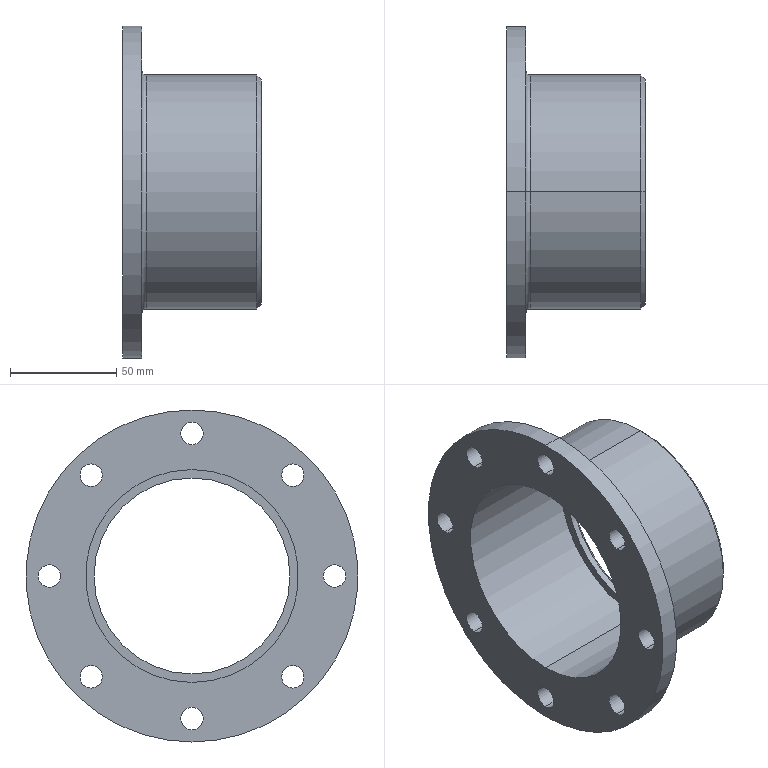Component | SolidWorks | UpperHousingAssembly-1_WormAxisAssembly-1_BearingSleeveOnWormAxis-1 | 1 solid | 34 faces | box 65 x 156 x 156 mm | volume 192466 mm3 | cylinder 24 | cone 4 | plane 4 | torus 2 | commonest cylinder face diameters 10.55 x16 92 x2 100 x2 110 x2 156 x2
build123d program:
from build123d import *

# Parameters (mm, degrees)
SKETCH1_R           = 78
BOSS_EXTRUDE1_DEPTH = 9
SKETCH2_R           = 55
BOSS_EXTRUDE2_DEPTH = 56
SKETCH3_R           = 50
CUT_EXTRUDE2_DEPTH  = 60
SKETCH4_R           = 46
CUT_EXTRUDE3_DEPTH  = 129.035
SKETCH5_R           = 5.275
CUT_EXTRUDE4_DEPTH  = 129.035
CIRPATTERN1_COUNT   = 8
CHAMFER1_SIZE       = 2
FILLET1_R           = 2


with BuildPart() as part:
    # Sketch1 → Boss-Extrude1 (new body)
    with BuildSketch(Plane.XY):
        Circle(SKETCH1_R)
    extrude(amount=BOSS_EXTRUDE1_DEPTH)

    # Sketch2 → Boss-Extrude2 (add)
    with BuildSketch(Plane.XY.offset(9)):
        Circle(SKETCH2_R)
    extrude(amount=BOSS_EXTRUDE2_DEPTH)

    # Sketch3 → Cut-Extrude2 (cut)
    with BuildSketch(Plane(origin=(0, 0, 0), x_dir=(-1, 0, 0), z_dir=(0, 0, -1))):
        Circle(SKETCH3_R)
    extrude(amount=-CUT_EXTRUDE2_DEPTH, mode=Mode.SUBTRACT)

    # Sketch4 → Cut-Extrude3 (cut, through all)
    with BuildSketch(Plane.XY.offset(65)):
        Circle(SKETCH4_R)
    extrude(amount=-CUT_EXTRUDE3_DEPTH, mode=Mode.SUBTRACT)

    # Sketch5 → Cut-Extrude4 (cut, through all)
    with BuildSketch(Plane(origin=(0, 0, 0), x_dir=(-1, 0, 0), z_dir=(0, 0, -1))):
        with Locations((0, 67)):
            Circle(SKETCH5_R)
    cut_extrude4 = extrude(amount=-CUT_EXTRUDE4_DEPTH, mode=Mode.SUBTRACT)

    # CirPattern1: Cut-Extrude4 ×8 about axis
    cirpattern1_axis = Axis((0, 0, 0), (0, 0, 1))
    for i in range(1, CIRPATTERN1_COUNT):
        add(cut_extrude4.rotate(cirpattern1_axis, i * 360 / CIRPATTERN1_COUNT), mode=Mode.SUBTRACT)

    # Chamfer1
    chamfer1_edges = [part.edges().sort_by_distance(p)[0] for p in [
        (-46, 0, 65),
        (-55, 0, 65),
    ]]
    chamfer(chamfer1_edges, length=CHAMFER1_SIZE)

    # Fillet1
    fillet1_edges = [part.edges().sort_by_distance(p)[0] for p in [
        (-55, 0, 9),
    ]]
    fillet(fillet1_edges, radius=FILLET1_R)


solid = part.part

# Placed as in the assembly
solid = solid.moved(Location((731.83, 1408.591, 1694.217), (0, 90, 0)))
STEP:
#1=COLOUR_RGB('',0.7922,0.8196,0.9333);
#2=FILL_AREA_STYLE_COLOUR('',#1);
#3=FILL_AREA_STYLE('',(#2));
#4=SURFACE_STYLE_FILL_AREA(#3);
#5=SURFACE_SIDE_STYLE('',(#4));
#6=SURFACE_STYLE_USAGE(.BOTH.,#5);
#7=PRESENTATION_STYLE_ASSIGNMENT((#6));
#8=CARTESIAN_POINT('',(29.245,55.456,68.867));
#9=VERTEX_POINT('',#8);
#10=CARTESIAN_POINT('',(29.245,55.456,64.536));
#11=VERTEX_POINT('',#10);
#12=CARTESIAN_POINT('',(29.245,55.456,66.701));
#13=DIRECTION('',(1.,0.,0.));
#14=DIRECTION('',(0.,0.,-1.));
#15=AXIS2_PLACEMENT_3D('',#12,#13,#14);
#16=CIRCLE('',#15,2.165);
#17=EDGE_CURVE('',#9,#11,#16,.T.);
#18=ORIENTED_EDGE('',*,*,#17,.F.);
#19=CARTESIAN_POINT('',(29.167,55.456,68.946));
#20=VERTEX_POINT('',#19);
#21=CARTESIAN_POINT('',(29.245,55.456,68.946));
#22=DIRECTION('',(-0.,1.,0.));
#23=DIRECTION('',(0.,0.,1.));
#24=AXIS2_PLACEMENT_3D('',#21,#22,#23);
#25=CIRCLE('',#24,0.07874);
#26=EDGE_CURVE('',#9,#20,#25,.T.);
#27=ORIENTED_EDGE('',*,*,#26,.T.);
#28=CARTESIAN_POINT('',(29.167,55.456,64.457));
#29=VERTEX_POINT('',#28);
#30=CARTESIAN_POINT('',(29.167,55.456,66.701));
#31=DIRECTION('',(-1.,-0.,-0.));
#32=DIRECTION('',(0.,0.,-1.));
#33=AXIS2_PLACEMENT_3D('',#30,#31,#32);
#34=CIRCLE('',#33,2.244);
#35=EDGE_CURVE('',#29,#20,#34,.T.);
#36=ORIENTED_EDGE('',*,*,#35,.F.);
#37=CARTESIAN_POINT('',(29.245,55.456,64.457));
#38=DIRECTION('',(0.,-1.,-0.));
#39=DIRECTION('',(0.,0.,-1.));
#40=AXIS2_PLACEMENT_3D('',#37,#38,#39);
#41=CIRCLE('',#40,0.07874);
#42=EDGE_CURVE('',#11,#29,#41,.T.);
#43=ORIENTED_EDGE('',*,*,#42,.F.);
#44=EDGE_LOOP('',(#18,#27,#36,#43));
#45=FACE_OUTER_BOUND('',#44,.T.);
#46=CARTESIAN_POINT('',(29.245,55.456,66.701));
#47=DIRECTION('',(1.,0.,0.));
#48=DIRECTION('',(0.,0.,-1.));
#49=AXIS2_PLACEMENT_3D('',#46,#47,#48);
#50=TOROIDAL_SURFACE('',#49,2.244,0.07874);
#51=ADVANCED_FACE('',(#45),#50,.F.);
#52=CARTESIAN_POINT('',(31.293,55.456,68.512));
#53=VERTEX_POINT('',#52);
#54=CARTESIAN_POINT('',(31.293,55.456,64.89));
#55=VERTEX_POINT('',#54);
#56=CARTESIAN_POINT('',(31.293,55.456,66.701));
#57=DIRECTION('',(1.,0.,0.));
#58=DIRECTION('',(0.,0.,-1.));
#59=AXIS2_PLACEMENT_3D('',#56,#57,#58);
#60=CIRCLE('',#59,1.811);
#61=EDGE_CURVE('',#53,#55,#60,.T.);
#62=ORIENTED_EDGE('',*,*,#61,.F.);
#63=CARTESIAN_POINT('',(31.371,55.456,68.591));
#64=VERTEX_POINT('',#63);
#65=CARTESIAN_POINT('',(31.293,55.456,68.512));
#66=DIRECTION('',(0.7071,-0.,0.7071));
#67=VECTOR('',#66,39.37);
#68=LINE('',#65,#67);
#69=EDGE_CURVE('',#53,#64,#68,.T.);
#70=ORIENTED_EDGE('',*,*,#69,.T.);
#71=CARTESIAN_POINT('',(31.371,55.456,64.812));
#72=VERTEX_POINT('',#71);
#73=CARTESIAN_POINT('',(31.371,55.456,66.701));
#74=DIRECTION('',(-1.,-0.,-0.));
#75=DIRECTION('',(0.,0.,-1.));
#76=AXIS2_PLACEMENT_3D('',#73,#74,#75);
#77=CIRCLE('',#76,1.89);
#78=EDGE_CURVE('',#72,#64,#77,.T.);
#79=ORIENTED_EDGE('',*,*,#78,.F.);
#80=CARTESIAN_POINT('',(31.293,55.456,64.89));
#81=DIRECTION('',(0.7071,0.,-0.7071));
#82=VECTOR('',#81,39.37);
#83=LINE('',#80,#82);
#84=EDGE_CURVE('',#55,#72,#83,.T.);
#85=ORIENTED_EDGE('',*,*,#84,.F.);
#86=EDGE_LOOP('',(#62,#70,#79,#85));
#87=FACE_OUTER_BOUND('',#86,.T.);
#88=CARTESIAN_POINT('',(31.293,55.456,66.701));
#89=DIRECTION('',(1.,0.,0.));
#90=DIRECTION('',(0.,0.,-1.));
#91=AXIS2_PLACEMENT_3D('',#88,#89,#90);
#92=CONICAL_SURFACE('',#91,1.811,0.7854);
#93=ADVANCED_FACE('',(#87),#92,.F.);
#94=CARTESIAN_POINT('',(31.371,55.456,64.615));
#95=VERTEX_POINT('',#94);
#96=CARTESIAN_POINT('',(31.371,55.456,68.788));
#97=VERTEX_POINT('',#96);
#98=CARTESIAN_POINT('',(31.371,55.456,66.701));
#99=DIRECTION('',(1.,0.,0.));
#100=DIRECTION('',(0.,0.,-1.));
#101=AXIS2_PLACEMENT_3D('',#98,#99,#100);
#102=CIRCLE('',#101,2.087);
#103=EDGE_CURVE('',#95,#97,#102,.T.);
#104=ORIENTED_EDGE('',*,*,#103,.F.);
#105=CARTESIAN_POINT('',(31.293,55.456,64.536));
#106=VERTEX_POINT('',#105);
#107=CARTESIAN_POINT('',(31.371,55.456,64.615));
#108=DIRECTION('',(-0.7071,0.,-0.7071));
#109=VECTOR('',#108,39.37);
#110=LINE('',#107,#109);
#111=EDGE_CURVE('',#95,#106,#110,.T.);
#112=ORIENTED_EDGE('',*,*,#111,.T.);
#113=CARTESIAN_POINT('',(31.293,55.456,68.867));
#114=VERTEX_POINT('',#113);
#115=CARTESIAN_POINT('',(31.293,55.456,66.701));
#116=DIRECTION('',(-1.,-0.,-0.));
#117=DIRECTION('',(0.,0.,-1.));
#118=AXIS2_PLACEMENT_3D('',#115,#116,#117);
#119=CIRCLE('',#118,2.165);
#120=EDGE_CURVE('',#114,#106,#119,.T.);
#121=ORIENTED_EDGE('',*,*,#120,.F.);
#122=CARTESIAN_POINT('',(31.371,55.456,68.788));
#123=DIRECTION('',(-0.7071,-0.,0.7071));
#124=VECTOR('',#123,39.37);
#125=LINE('',#122,#124);
#126=EDGE_CURVE('',#97,#114,#125,.T.);
#127=ORIENTED_EDGE('',*,*,#126,.F.);
#128=EDGE_LOOP('',(#104,#112,#121,#127));
#129=FACE_OUTER_BOUND('',#128,.T.);
#130=CARTESIAN_POINT('',(31.371,55.456,66.701));
#131=DIRECTION('',(-1.,-0.,-0.));
#132=DIRECTION('',(0.,0.,1.));
#133=AXIS2_PLACEMENT_3D('',#130,#131,#132);
#134=CONICAL_SURFACE('',#133,2.087,0.7854);
#135=ADVANCED_FACE('',(#129),#134,.T.);
#136=CARTESIAN_POINT('',(29.167,55.456,64.271));
#137=VERTEX_POINT('',#136);
#138=CARTESIAN_POINT('',(29.167,55.456,63.856));
#139=VERTEX_POINT('',#138);
#140=CARTESIAN_POINT('',(29.167,55.456,64.064));
#141=DIRECTION('',(1.,0.,0.));
#142=DIRECTION('',(0.,0.,-1.));
#143=AXIS2_PLACEMENT_3D('',#140,#141,#142);
#144=CIRCLE('',#143,0.2077);
#145=EDGE_CURVE('',#137,#139,#144,.T.);
#146=ORIENTED_EDGE('',*,*,#145,.T.);
#147=CARTESIAN_POINT('',(28.812,55.456,63.856));
#148=VERTEX_POINT('',#147);
#149=CARTESIAN_POINT('',(31.371,55.456,63.856));
#150=DIRECTION('',(-1.,-0.,-0.));
#151=VECTOR('',#150,39.37);
#152=LINE('',#149,#151);
#153=EDGE_CURVE('',#139,#148,#152,.T.);
#154=ORIENTED_EDGE('',*,*,#153,.T.);
#155=CARTESIAN_POINT('',(28.812,55.456,64.271));
#156=VERTEX_POINT('',#155);
#157=CARTESIAN_POINT('',(28.812,55.456,64.064));
#158=DIRECTION('',(-1.,-0.,-0.));
#159=DIRECTION('',(0.,1.,0.));
#160=AXIS2_PLACEMENT_3D('',#157,#158,#159);
#161=CIRCLE('',#160,0.2077);
#162=EDGE_CURVE('',#148,#156,#161,.T.);
#163=ORIENTED_EDGE('',*,*,#162,.T.);
#164=CARTESIAN_POINT('',(31.371,55.456,64.271));
#165=DIRECTION('',(-1.,-0.,-0.));
#166=VECTOR('',#165,39.37);
#167=LINE('',#164,#166);
#168=EDGE_CURVE('',#137,#156,#167,.T.);
#169=ORIENTED_EDGE('',*,*,#168,.F.);
#170=EDGE_LOOP('',(#146,#154,#163,#169));
#171=FACE_OUTER_BOUND('',#170,.T.);
#172=CARTESIAN_POINT('',(31.371,55.456,64.064));
#173=DIRECTION('',(-1.,-0.,-0.));
#174=DIRECTION('',(0.,0.,1.));
#175=AXIS2_PLACEMENT_3D('',#172,#173,#174);
#176=CYLINDRICAL_SURFACE('',#175,0.2077);
#177=ADVANCED_FACE('',(#171),#176,.F.);
#178=CARTESIAN_POINT('',(29.167,53.591,65.044));
#179=VERTEX_POINT('',#178);
#180=CARTESIAN_POINT('',(29.167,53.591,64.629));
#181=VERTEX_POINT('',#180);
#182=CARTESIAN_POINT('',(29.167,53.591,64.836));
#183=DIRECTION('',(1.,0.,0.));
#184=DIRECTION('',(0.,0.,-1.));
#185=AXIS2_PLACEMENT_3D('',#182,#183,#184);
#186=CIRCLE('',#185,0.2077);
#187=EDGE_CURVE('',#179,#181,#186,.T.);
#188=ORIENTED_EDGE('',*,*,#187,.T.);
#189=CARTESIAN_POINT('',(28.812,53.591,64.629));
#190=VERTEX_POINT('',#189);
#191=CARTESIAN_POINT('',(31.371,53.591,64.629));
#192=DIRECTION('',(-1.,-0.,-0.));
#193=VECTOR('',#192,39.37);
#194=LINE('',#191,#193);
#195=EDGE_CURVE('',#181,#190,#194,.T.);
#196=ORIENTED_EDGE('',*,*,#195,.T.);
#197=CARTESIAN_POINT('',(28.812,53.591,65.044));
#198=VERTEX_POINT('',#197);
#199=CARTESIAN_POINT('',(28.812,53.591,64.836));
#200=DIRECTION('',(-1.,-0.,-0.));
#201=DIRECTION('',(0.,0.7071,-0.7071));
#202=AXIS2_PLACEMENT_3D('',#199,#200,#201);
#203=CIRCLE('',#202,0.2077);
#204=EDGE_CURVE('',#190,#198,#203,.T.);
#205=ORIENTED_EDGE('',*,*,#204,.T.);
#206=CARTESIAN_POINT('',(31.371,53.591,65.044));
#207=DIRECTION('',(-1.,-0.,-0.));
#208=VECTOR('',#207,39.37);
#209=LINE('',#206,#208);
#210=EDGE_CURVE('',#179,#198,#209,.T.);
#211=ORIENTED_EDGE('',*,*,#210,.F.);
#212=EDGE_LOOP('',(#188,#196,#205,#211));
#213=FACE_OUTER_BOUND('',#212,.T.);
#214=CARTESIAN_POINT('',(31.371,53.591,64.836));
#215=DIRECTION('',(-1.,-0.,-0.));
#216=DIRECTION('',(0.,0.,1.));
#217=AXIS2_PLACEMENT_3D('',#214,#215,#216);
#218=CYLINDRICAL_SURFACE('',#217,0.2077);
#219=ADVANCED_FACE('',(#213),#218,.F.);
#220=CARTESIAN_POINT('',(29.167,52.819,66.909));
#221=VERTEX_POINT('',#220);
#222=CARTESIAN_POINT('',(29.167,52.819,66.494));
#223=VERTEX_POINT('',#222);
#224=CARTESIAN_POINT('',(29.167,52.819,66.701));
#225=DIRECTION('',(1.,0.,0.));
#226=DIRECTION('',(0.,0.,-1.));
#227=AXIS2_PLACEMENT_3D('',#224,#225,#226);
#228=CIRCLE('',#227,0.2077);
#229=EDGE_CURVE('',#221,#223,#228,.T.);
#230=ORIENTED_EDGE('',*,*,#229,.T.);
#231=CARTESIAN_POINT('',(28.812,52.819,66.494));
#232=VERTEX_POINT('',#231);
#233=CARTESIAN_POINT('',(31.371,52.819,66.494));
#234=DIRECTION('',(-1.,-0.,-0.));
#235=VECTOR('',#234,39.37);
#236=LINE('',#233,#235);
#237=EDGE_CURVE('',#223,#232,#236,.T.);
#238=ORIENTED_EDGE('',*,*,#237,.T.);
#239=CARTESIAN_POINT('',(28.812,52.819,66.909));
#240=VERTEX_POINT('',#239);
#241=CARTESIAN_POINT('',(28.812,52.819,66.701));
#242=DIRECTION('',(-1.,-0.,-0.));
#243=DIRECTION('',(0.,0.,-1.));
#244=AXIS2_PLACEMENT_3D('',#241,#242,#243);
#245=CIRCLE('',#244,0.2077);
#246=EDGE_CURVE('',#232,#240,#245,.T.);
#247=ORIENTED_EDGE('',*,*,#246,.T.);
#248=CARTESIAN_POINT('',(31.371,52.819,66.909));
#249=DIRECTION('',(-1.,-0.,-0.));
#250=VECTOR('',#249,39.37);
#251=LINE('',#248,#250);
#252=EDGE_CURVE('',#221,#240,#251,.T.);
#253=ORIENTED_EDGE('',*,*,#252,.F.);
#254=EDGE_LOOP('',(#230,#238,#247,#253));
#255=FACE_OUTER_BOUND('',#254,.T.);
#256=CARTESIAN_POINT('',(31.371,52.819,66.701));
#257=DIRECTION('',(-1.,-0.,-0.));
#258=DIRECTION('',(0.,0.,1.));
#259=AXIS2_PLACEMENT_3D('',#256,#257,#258);
#260=CYLINDRICAL_SURFACE('',#259,0.2077);
#261=ADVANCED_FACE('',(#255),#260,.F.);
#262=CARTESIAN_POINT('',(29.167,53.591,68.774));
#263=VERTEX_POINT('',#262);
#264=CARTESIAN_POINT('',(29.167,53.591,68.359));
#265=VERTEX_POINT('',#264);
#266=CARTESIAN_POINT('',(29.167,53.591,68.567));
#267=DIRECTION('',(1.,0.,0.));
#268=DIRECTION('',(0.,0.,-1.));
#269=AXIS2_PLACEMENT_3D('',#266,#267,#268);
#270=CIRCLE('',#269,0.2077);
#271=EDGE_CURVE('',#263,#265,#270,.T.);
#272=ORIENTED_EDGE('',*,*,#271,.T.);
#273=CARTESIAN_POINT('',(28.812,53.591,68.359));
#274=VERTEX_POINT('',#273);
#275=CARTESIAN_POINT('',(31.371,53.591,68.359));
#276=DIRECTION('',(-1.,-0.,-0.));
#277=VECTOR('',#276,39.37);
#278=LINE('',#275,#277);
#279=EDGE_CURVE('',#265,#274,#278,.T.);
#280=ORIENTED_EDGE('',*,*,#279,.T.);
#281=CARTESIAN_POINT('',(28.812,53.591,68.774));
#282=VERTEX_POINT('',#281);
#283=CARTESIAN_POINT('',(28.812,53.591,68.567));
#284=DIRECTION('',(-1.,-0.,-0.));
#285=DIRECTION('',(0.,-0.7071,-0.7071));
#286=AXIS2_PLACEMENT_3D('',#283,#284,#285);
#287=CIRCLE('',#286,0.2077);
#288=EDGE_CURVE('',#274,#282,#287,.T.);
#289=ORIENTED_EDGE('',*,*,#288,.T.);
#290=CARTESIAN_POINT('',(31.371,53.591,68.774));
#291=DIRECTION('',(-1.,-0.,-0.));
#292=VECTOR('',#291,39.37);
#293=LINE('',#290,#292);
#294=EDGE_CURVE('',#263,#282,#293,.T.);
#295=ORIENTED_EDGE('',*,*,#294,.F.);
#296=EDGE_LOOP('',(#272,#280,#289,#295));
#297=FACE_OUTER_BOUND('',#296,.T.);
#298=CARTESIAN_POINT('',(31.371,53.591,68.567));
#299=DIRECTION('',(-1.,-0.,-0.));
#300=DIRECTION('',(0.,0.,1.));
#301=AXIS2_PLACEMENT_3D('',#298,#299,#300);
#302=CYLINDRICAL_SURFACE('',#301,0.2077);
#303=ADVANCED_FACE('',(#297),#302,.F.);
#304=CARTESIAN_POINT('',(29.167,55.456,69.547));
#305=VERTEX_POINT('',#304);
#306=CARTESIAN_POINT('',(29.167,55.456,69.132));
#307=VERTEX_POINT('',#306);
#308=CARTESIAN_POINT('',(29.167,55.456,69.339));
#309=DIRECTION('',(1.,0.,0.));
#310=DIRECTION('',(0.,0.,-1.));
#311=AXIS2_PLACEMENT_3D('',#308,#309,#310);
#312=CIRCLE('',#311,0.2077);
#313=EDGE_CURVE('',#305,#307,#312,.T.);
#314=ORIENTED_EDGE('',*,*,#313,.T.);
#315=CARTESIAN_POINT('',(28.812,55.456,69.132));
#316=VERTEX_POINT('',#315);
#317=CARTESIAN_POINT('',(31.371,55.456,69.132));
#318=DIRECTION('',(-1.,-0.,-0.));
#319=VECTOR('',#318,39.37);
#320=LINE('',#317,#319);
#321=EDGE_CURVE('',#307,#316,#320,.T.);
#322=ORIENTED_EDGE('',*,*,#321,.T.);
#323=CARTESIAN_POINT('',(28.812,55.456,69.547));
#324=VERTEX_POINT('',#323);
#325=CARTESIAN_POINT('',(28.812,55.456,69.339));
#326=DIRECTION('',(-1.,-0.,-0.));
#327=DIRECTION('',(0.,-1.,0.));
#328=AXIS2_PLACEMENT_3D('',#325,#326,#327);
#329=CIRCLE('',#328,0.2077);
#330=EDGE_CURVE('',#316,#324,#329,.T.);
#331=ORIENTED_EDGE('',*,*,#330,.T.);
#332=CARTESIAN_POINT('',(31.371,55.456,69.547));
#333=DIRECTION('',(-1.,-0.,-0.));
#334=VECTOR('',#333,39.37);
#335=LINE('',#332,#334);
#336=EDGE_CURVE('',#305,#324,#335,.T.);
#337=ORIENTED_EDGE('',*,*,#336,.F.);
#338=EDGE_LOOP('',(#314,#322,#331,#337));
#339=FACE_OUTER_BOUND('',#338,.T.);
#340=CARTESIAN_POINT('',(31.371,55.456,69.339));
#341=DIRECTION('',(-1.,-0.,-0.));
#342=DIRECTION('',(0.,0.,1.));
#343=AXIS2_PLACEMENT_3D('',#340,#341,#342);
#344=CYLINDRICAL_SURFACE('',#343,0.2077);
#345=ADVANCED_FACE('',(#339),#344,.F.);
#346=CARTESIAN_POINT('',(29.167,57.322,68.774));
#347=VERTEX_POINT('',#346);
#348=CARTESIAN_POINT('',(29.167,57.322,68.359));
#349=VERTEX_POINT('',#348);
#350=CARTESIAN_POINT('',(29.167,57.322,68.567));
#351=DIRECTION('',(1.,0.,0.));
#352=DIRECTION('',(0.,0.,-1.));
#353=AXIS2_PLACEMENT_3D('',#350,#351,#352);
#354=CIRCLE('',#353,0.2077);
#355=EDGE_CURVE('',#347,#349,#354,.T.);
#356=ORIENTED_EDGE('',*,*,#355,.T.);
#357=CARTESIAN_POINT('',(28.812,57.322,68.359));
#358=VERTEX_POINT('',#357);
#359=CARTESIAN_POINT('',(31.371,57.322,68.359));
#360=DIRECTION('',(-1.,-0.,-0.));
#361=VECTOR('',#360,39.37);
#362=LINE('',#359,#361);
#363=EDGE_CURVE('',#349,#358,#362,.T.);
#364=ORIENTED_EDGE('',*,*,#363,.T.);
#365=CARTESIAN_POINT('',(28.812,57.322,68.774));
#366=VERTEX_POINT('',#365);
#367=CARTESIAN_POINT('',(28.812,57.322,68.567));
#368=DIRECTION('',(-1.,-0.,-0.));
#369=DIRECTION('',(0.,-0.7071,0.7071));
#370=AXIS2_PLACEMENT_3D('',#367,#368,#369);
#371=CIRCLE('',#370,0.2077);
#372=EDGE_CURVE('',#358,#366,#371,.T.);
#373=ORIENTED_EDGE('',*,*,#372,.T.);
#374=CARTESIAN_POINT('',(31.371,57.322,68.774));
#375=DIRECTION('',(-1.,-0.,-0.));
#376=VECTOR('',#375,39.37);
#377=LINE('',#374,#376);
#378=EDGE_CURVE('',#347,#366,#377,.T.);
#379=ORIENTED_EDGE('',*,*,#378,.F.);
#380=EDGE_LOOP('',(#356,#364,#373,#379));
#381=FACE_OUTER_BOUND('',#380,.T.);
#382=CARTESIAN_POINT('',(31.371,57.322,68.567));
#383=DIRECTION('',(-1.,-0.,-0.));
#384=DIRECTION('',(0.,0.,1.));
#385=AXIS2_PLACEMENT_3D('',#382,#383,#384);
#386=CYLINDRICAL_SURFACE('',#385,0.2077);
#387=ADVANCED_FACE('',(#381),#386,.F.);
#388=CARTESIAN_POINT('',(29.167,57.322,65.044));
#389=VERTEX_POINT('',#388);
#390=CARTESIAN_POINT('',(29.167,57.322,64.629));
#391=VERTEX_POINT('',#390);
#392=CARTESIAN_POINT('',(29.167,57.322,64.836));
#393=DIRECTION('',(1.,0.,0.));
#394=DIRECTION('',(0.,0.,-1.));
#395=AXIS2_PLACEMENT_3D('',#392,#393,#394);
#396=CIRCLE('',#395,0.2077);
#397=EDGE_CURVE('',#389,#391,#396,.T.);
#398=ORIENTED_EDGE('',*,*,#397,.T.);
#399=CARTESIAN_POINT('',(28.812,57.322,64.629));
#400=VERTEX_POINT('',#399);
#401=CARTESIAN_POINT('',(31.371,57.322,64.629));
#402=DIRECTION('',(-1.,-0.,-0.));
#403=VECTOR('',#402,39.37);
#404=LINE('',#401,#403);
#405=EDGE_CURVE('',#391,#400,#404,.T.);
#406=ORIENTED_EDGE('',*,*,#405,.T.);
#407=CARTESIAN_POINT('',(28.812,57.322,65.044));
#408=VERTEX_POINT('',#407);
#409=CARTESIAN_POINT('',(28.812,57.322,64.836));
#410=DIRECTION('',(-1.,-0.,-0.));
#411=DIRECTION('',(0.,0.7071,0.7071));
#412=AXIS2_PLACEMENT_3D('',#409,#410,#411);
#413=CIRCLE('',#412,0.2077);
#414=EDGE_CURVE('',#400,#408,#413,.T.);
#415=ORIENTED_EDGE('',*,*,#414,.T.);
#416=CARTESIAN_POINT('',(31.371,57.322,65.044));
#417=DIRECTION('',(-1.,-0.,-0.));
#418=VECTOR('',#417,39.37);
#419=LINE('',#416,#418);
#420=EDGE_CURVE('',#389,#408,#419,.T.);
#421=ORIENTED_EDGE('',*,*,#420,.F.);
#422=EDGE_LOOP('',(#398,#406,#415,#421));
#423=FACE_OUTER_BOUND('',#422,.T.);
#424=CARTESIAN_POINT('',(31.371,57.322,64.836));
#425=DIRECTION('',(-1.,-0.,-0.));
#426=DIRECTION('',(0.,0.,1.));
#427=AXIS2_PLACEMENT_3D('',#424,#425,#426);
#428=CYLINDRICAL_SURFACE('',#427,0.2077);
#429=ADVANCED_FACE('',(#423),#428,.F.);
#430=CARTESIAN_POINT('',(29.167,58.094,66.909));
#431=VERTEX_POINT('',#430);
#432=CARTESIAN_POINT('',(29.167,58.094,66.494));
#433=VERTEX_POINT('',#432);
#434=CARTESIAN_POINT('',(29.167,58.094,66.701));
#435=DIRECTION('',(1.,0.,0.));
#436=DIRECTION('',(0.,0.,-1.));
#437=AXIS2_PLACEMENT_3D('',#434,#435,#436);
#438=CIRCLE('',#437,0.2077);
#439=EDGE_CURVE('',#431,#433,#438,.T.);
#440=ORIENTED_EDGE('',*,*,#439,.T.);
#441=CARTESIAN_POINT('',(28.812,58.094,66.494));
#442=VERTEX_POINT('',#441);
#443=CARTESIAN_POINT('',(31.371,58.094,66.494));
#444=DIRECTION('',(-1.,-0.,-0.));
#445=VECTOR('',#444,39.37);
#446=LINE('',#443,#445);
#447=EDGE_CURVE('',#433,#442,#446,.T.);
#448=ORIENTED_EDGE('',*,*,#447,.T.);
#449=CARTESIAN_POINT('',(28.812,58.094,66.909));
#450=VERTEX_POINT('',#449);
#451=CARTESIAN_POINT('',(28.812,58.094,66.701));
#452=DIRECTION('',(-1.,-0.,-0.));
#453=DIRECTION('',(0.,0.,1.));
#454=AXIS2_PLACEMENT_3D('',#451,#452,#453);
#455=CIRCLE('',#454,0.2077);
#456=EDGE_CURVE('',#442,#450,#455,.T.);
#457=ORIENTED_EDGE('',*,*,#456,.T.);
#458=CARTESIAN_POINT('',(31.371,58.094,66.909));
#459=DIRECTION('',(-1.,-0.,-0.));
#460=VECTOR('',#459,39.37);
#461=LINE('',#458,#460);
#462=EDGE_CURVE('',#431,#450,#461,.T.);
#463=ORIENTED_EDGE('',*,*,#462,.F.);
#464=EDGE_LOOP('',(#440,#448,#457,#463));
#465=FACE_OUTER_BOUND('',#464,.T.);
#466=CARTESIAN_POINT('',(31.371,58.094,66.701));
#467=DIRECTION('',(-1.,-0.,-0.));
#468=DIRECTION('',(0.,0.,1.));
#469=AXIS2_PLACEMENT_3D('',#466,#467,#468);
#470=CYLINDRICAL_SURFACE('',#469,0.2077);
#471=ADVANCED_FACE('',(#465),#470,.F.);
#472=CARTESIAN_POINT('',(31.174,55.456,64.89));
#473=VERTEX_POINT('',#472);
#474=CARTESIAN_POINT('',(31.174,55.456,68.512));
#475=VERTEX_POINT('',#474);
#476=CARTESIAN_POINT('',(31.174,55.456,66.701));
#477=DIRECTION('',(-1.,-0.,-0.));
#478=DIRECTION('',(0.,0.,1.));
#479=AXIS2_PLACEMENT_3D('',#476,#477,#478);
#480=CIRCLE('',#479,1.811);
#481=EDGE_CURVE('',#473,#475,#480,.T.);
#482=ORIENTED_EDGE('',*,*,#481,.T.);
#483=CARTESIAN_POINT('',(28.812,55.456,68.512));
#484=DIRECTION('',(1.,0.,0.));
#485=VECTOR('',#484,39.37);
#486=LINE('',#483,#485);
#487=EDGE_CURVE('',#475,#53,#486,.T.);
#488=ORIENTED_EDGE('',*,*,#487,.T.);
#489=ORIENTED_EDGE('',*,*,#61,.T.);
#490=CARTESIAN_POINT('',(28.812,55.456,64.89));
#491=DIRECTION('',(1.,0.,0.));
#492=VECTOR('',#491,39.37);
#493=LINE('',#490,#492);
#494=EDGE_CURVE('',#473,#55,#493,.T.);
#495=ORIENTED_EDGE('',*,*,#494,.F.);
#496=EDGE_LOOP('',(#482,#488,#489,#495));
#497=FACE_OUTER_BOUND('',#496,.T.);
#498=CARTESIAN_POINT('',(28.812,55.456,66.701));
#499=DIRECTION('',(1.,0.,0.));
#500=DIRECTION('',(0.,0.,-1.));
#501=AXIS2_PLACEMENT_3D('',#498,#499,#500);
#502=CYLINDRICAL_SURFACE('',#501,1.811);
#503=ADVANCED_FACE('',(#497),#502,.F.);
#504=CARTESIAN_POINT('',(31.174,55.456,64.733));
#505=VERTEX_POINT('',#504);
#506=CARTESIAN_POINT('',(31.174,55.456,68.67));
#507=VERTEX_POINT('',#506);
#508=CARTESIAN_POINT('',(31.174,55.456,66.701));
#509=DIRECTION('',(-1.,-0.,-0.));
#510=DIRECTION('',(0.,0.,1.));
#511=AXIS2_PLACEMENT_3D('',#508,#509,#510);
#512=CIRCLE('',#511,1.969);
#513=EDGE_CURVE('',#505,#507,#512,.T.);
#514=ORIENTED_EDGE('',*,*,#513,.F.);
#515=CARTESIAN_POINT('',(28.812,55.456,64.733));
#516=VERTEX_POINT('',#515);
#517=CARTESIAN_POINT('',(31.174,55.456,64.733));
#518=DIRECTION('',(-1.,-0.,-0.));
#519=VECTOR('',#518,39.37);
#520=LINE('',#517,#519);
#521=EDGE_CURVE('',#505,#516,#520,.T.);
#522=ORIENTED_EDGE('',*,*,#521,.T.);
#523=CARTESIAN_POINT('',(28.812,55.456,68.67));
#524=VERTEX_POINT('',#523);
#525=CARTESIAN_POINT('',(28.812,55.456,66.701));
#526=DIRECTION('',(-1.,-0.,-0.));
#527=DIRECTION('',(0.,0.,1.));
#528=AXIS2_PLACEMENT_3D('',#525,#526,#527);
#529=CIRCLE('',#528,1.969);
#530=EDGE_CURVE('',#516,#524,#529,.T.);
#531=ORIENTED_EDGE('',*,*,#530,.T.);
#532=CARTESIAN_POINT('',(31.174,55.456,68.67));
#533=DIRECTION('',(-1.,-0.,-0.));
#534=VECTOR('',#533,39.37);
#535=LINE('',#532,#534);
#536=EDGE_CURVE('',#507,#524,#535,.T.);
#537=ORIENTED_EDGE('',*,*,#536,.F.);
#538=EDGE_LOOP('',(#514,#522,#531,#537));
#539=FACE_OUTER_BOUND('',#538,.T.);
#540=CARTESIAN_POINT('',(31.174,55.456,66.701));
#541=DIRECTION('',(-1.,-0.,-0.));
#542=DIRECTION('',(0.,0.,1.));
#543=AXIS2_PLACEMENT_3D('',#540,#541,#542);
#544=CYLINDRICAL_SURFACE('',#543,1.969);
#545=ADVANCED_FACE('',(#539),#544,.F.);
#546=ORIENTED_EDGE('',*,*,#120,.T.);
#547=CARTESIAN_POINT('',(31.371,55.456,64.536));
#548=DIRECTION('',(-1.,-0.,-0.));
#549=VECTOR('',#548,39.37);
#550=LINE('',#547,#549);
#551=EDGE_CURVE('',#106,#11,#550,.T.);
#552=ORIENTED_EDGE('',*,*,#551,.T.);
#553=CARTESIAN_POINT('',(29.245,55.456,66.701));
#554=DIRECTION('',(1.,0.,0.));
#555=DIRECTION('',(0.,0.,-1.));
#556=AXIS2_PLACEMENT_3D('',#553,#554,#555);
#557=CIRCLE('',#556,2.165);
#558=EDGE_CURVE('',#11,#9,#557,.T.);
#559=ORIENTED_EDGE('',*,*,#558,.T.);
#560=CARTESIAN_POINT('',(31.371,55.456,68.867));
#561=DIRECTION('',(-1.,-0.,-0.));
#562=VECTOR('',#561,39.37);
#563=LINE('',#560,#562);
#564=EDGE_CURVE('',#114,#9,#563,.T.);
#565=ORIENTED_EDGE('',*,*,#564,.F.);
#566=EDGE_LOOP('',(#546,#552,#559,#565));
#567=FACE_OUTER_BOUND('',#566,.T.);
#568=CARTESIAN_POINT('',(31.371,55.456,66.701));
#569=DIRECTION('',(-1.,-0.,-0.));
#570=DIRECTION('',(0.,0.,1.));
#571=AXIS2_PLACEMENT_3D('',#568,#569,#570);
#572=CYLINDRICAL_SURFACE('',#571,2.165);
#573=ADVANCED_FACE('',(#567),#572,.T.);
#574=CARTESIAN_POINT('',(29.167,55.456,63.631));
#575=VERTEX_POINT('',#574);
#576=CARTESIAN_POINT('',(29.167,55.456,69.772));
#577=VERTEX_POINT('',#576);
#578=CARTESIAN_POINT('',(29.167,55.456,66.701));
#579=DIRECTION('',(1.,0.,0.));
#580=DIRECTION('',(0.,0.,-1.));
#581=AXIS2_PLACEMENT_3D('',#578,#579,#580);
#582=CIRCLE('',#581,3.071);
#583=EDGE_CURVE('',#575,#577,#582,.T.);
#584=ORIENTED_EDGE('',*,*,#583,.F.);
#585=CARTESIAN_POINT('',(28.812,55.456,63.631));
#586=VERTEX_POINT('',#585);
#587=CARTESIAN_POINT('',(29.167,55.456,63.631));
#588=DIRECTION('',(-1.,-0.,-0.));
#589=VECTOR('',#588,39.37);
#590=LINE('',#587,#589);
#591=EDGE_CURVE('',#575,#586,#590,.T.);
#592=ORIENTED_EDGE('',*,*,#591,.T.);
#593=CARTESIAN_POINT('',(28.812,55.456,69.772));
#594=VERTEX_POINT('',#593);
#595=CARTESIAN_POINT('',(28.812,55.456,66.701));
#596=DIRECTION('',(1.,0.,0.));
#597=DIRECTION('',(0.,0.,-1.));
#598=AXIS2_PLACEMENT_3D('',#595,#596,#597);
#599=CIRCLE('',#598,3.071);
#600=EDGE_CURVE('',#586,#594,#599,.T.);
#601=ORIENTED_EDGE('',*,*,#600,.T.);
#602=CARTESIAN_POINT('',(29.167,55.456,69.772));
#603=DIRECTION('',(-1.,-0.,-0.));
#604=VECTOR('',#603,39.37);
#605=LINE('',#602,#604);
#606=EDGE_CURVE('',#577,#594,#605,.T.);
#607=ORIENTED_EDGE('',*,*,#606,.F.);
#608=EDGE_LOOP('',(#584,#592,#601,#607));
#609=FACE_OUTER_BOUND('',#608,.T.);
#610=CARTESIAN_POINT('',(29.167,55.456,66.701));
#611=DIRECTION('',(-1.,-0.,-0.));
#612=DIRECTION('',(0.,-0.,1.));
#613=AXIS2_PLACEMENT_3D('',#610,#611,#612);
#614=CYLINDRICAL_SURFACE('',#613,3.071);
#615=ADVANCED_FACE('',(#609),#614,.T.);
#616=ORIENTED_EDGE('',*,*,#591,.F.);
#617=CARTESIAN_POINT('',(29.167,55.456,66.701));
#618=DIRECTION('',(1.,0.,0.));
#619=DIRECTION('',(0.,0.,-1.));
#620=AXIS2_PLACEMENT_3D('',#617,#618,#619);
#621=CIRCLE('',#620,3.071);
#622=EDGE_CURVE('',#577,#575,#621,.T.);
#623=ORIENTED_EDGE('',*,*,#622,.F.);
#624=ORIENTED_EDGE('',*,*,#606,.T.);
#625=CARTESIAN_POINT('',(28.812,55.456,66.701));
#626=DIRECTION('',(1.,0.,0.));
#627=DIRECTION('',(0.,0.,-1.));
#628=AXIS2_PLACEMENT_3D('',#625,#626,#627);
#629=CIRCLE('',#628,3.071);
#630=EDGE_CURVE('',#594,#586,#629,.T.);
#631=ORIENTED_EDGE('',*,*,#630,.T.);
#632=EDGE_LOOP('',(#616,#623,#624,#631));
#633=FACE_OUTER_BOUND('',#632,.T.);
#634=CARTESIAN_POINT('',(29.167,55.456,66.701));
#635=DIRECTION('',(-1.,-0.,-0.));
#636=DIRECTION('',(0.,-0.,1.));
#637=AXIS2_PLACEMENT_3D('',#634,#635,#636);
#638=CYLINDRICAL_SURFACE('',#637,3.071);
#639=ADVANCED_FACE('',(#633),#638,.T.);
#640=ORIENTED_EDGE('',*,*,#35,.T.);
#641=CARTESIAN_POINT('',(29.167,55.456,66.701));
#642=DIRECTION('',(-1.,-0.,-0.));
#643=DIRECTION('',(0.,0.,-1.));
#644=AXIS2_PLACEMENT_3D('',#641,#642,#643);
#645=CIRCLE('',#644,2.244);
#646=EDGE_CURVE('',#20,#29,#645,.T.);
#647=ORIENTED_EDGE('',*,*,#646,.T.);
#648=EDGE_LOOP('',(#640,#647));
#649=FACE_BOUND('',#648,.T.);
#650=ORIENTED_EDGE('',*,*,#145,.F.);
#651=CARTESIAN_POINT('',(29.167,55.456,64.064));
#652=DIRECTION('',(1.,0.,0.));
#653=DIRECTION('',(0.,0.,-1.));
#654=AXIS2_PLACEMENT_3D('',#651,#652,#653);
#655=CIRCLE('',#654,0.2077);
#656=EDGE_CURVE('',#139,#137,#655,.T.);
#657=ORIENTED_EDGE('',*,*,#656,.F.);
#658=EDGE_LOOP('',(#650,#657));
#659=FACE_BOUND('',#658,.T.);
#660=ORIENTED_EDGE('',*,*,#187,.F.);
#661=CARTESIAN_POINT('',(29.167,53.591,64.836));
#662=DIRECTION('',(1.,0.,0.));
#663=DIRECTION('',(0.,0.,-1.));
#664=AXIS2_PLACEMENT_3D('',#661,#662,#663);
#665=CIRCLE('',#664,0.2077);
#666=EDGE_CURVE('',#181,#179,#665,.T.);
#667=ORIENTED_EDGE('',*,*,#666,.F.);
#668=EDGE_LOOP('',(#660,#667));
#669=FACE_BOUND('',#668,.T.);
#670=ORIENTED_EDGE('',*,*,#229,.F.);
#671=CARTESIAN_POINT('',(29.167,52.819,66.701));
#672=DIRECTION('',(1.,0.,0.));
#673=DIRECTION('',(0.,0.,-1.));
#674=AXIS2_PLACEMENT_3D('',#671,#672,#673);
#675=CIRCLE('',#674,0.2077);
#676=EDGE_CURVE('',#223,#221,#675,.T.);
#677=ORIENTED_EDGE('',*,*,#676,.F.);
#678=EDGE_LOOP('',(#670,#677));
#679=FACE_BOUND('',#678,.T.);
#680=ORIENTED_EDGE('',*,*,#271,.F.);
#681=CARTESIAN_POINT('',(29.167,53.591,68.567));
#682=DIRECTION('',(1.,0.,0.));
#683=DIRECTION('',(0.,0.,-1.));
#684=AXIS2_PLACEMENT_3D('',#681,#682,#683);
#685=CIRCLE('',#684,0.2077);
#686=EDGE_CURVE('',#265,#263,#685,.T.);
#687=ORIENTED_EDGE('',*,*,#686,.F.);
#688=EDGE_LOOP('',(#680,#687));
#689=FACE_BOUND('',#688,.T.);
#690=ORIENTED_EDGE('',*,*,#313,.F.);
#691=CARTESIAN_POINT('',(29.167,55.456,69.339));
#692=DIRECTION('',(1.,0.,0.));
#693=DIRECTION('',(0.,0.,-1.));
#694=AXIS2_PLACEMENT_3D('',#691,#692,#693);
#695=CIRCLE('',#694,0.2077);
#696=EDGE_CURVE('',#307,#305,#695,.T.);
#697=ORIENTED_EDGE('',*,*,#696,.F.);
#698=EDGE_LOOP('',(#690,#697));
#699=FACE_BOUND('',#698,.T.);
#700=ORIENTED_EDGE('',*,*,#355,.F.);
#701=CARTESIAN_POINT('',(29.167,57.322,68.567));
#702=DIRECTION('',(1.,0.,0.));
#703=DIRECTION('',(0.,0.,-1.));
#704=AXIS2_PLACEMENT_3D('',#701,#702,#703);
#705=CIRCLE('',#704,0.2077);
#706=EDGE_CURVE('',#349,#347,#705,.T.);
#707=ORIENTED_EDGE('',*,*,#706,.F.);
#708=EDGE_LOOP('',(#700,#707));
#709=FACE_BOUND('',#708,.T.);
#710=ORIENTED_EDGE('',*,*,#397,.F.);
#711=CARTESIAN_POINT('',(29.167,57.322,64.836));
#712=DIRECTION('',(1.,0.,0.));
#713=DIRECTION('',(0.,0.,-1.));
#714=AXIS2_PLACEMENT_3D('',#711,#712,#713);
#715=CIRCLE('',#714,0.2077);
#716=EDGE_CURVE('',#391,#389,#715,.T.);
#717=ORIENTED_EDGE('',*,*,#716,.F.);
#718=EDGE_LOOP('',(#710,#717));
#719=FACE_BOUND('',#718,.T.);
#720=ORIENTED_EDGE('',*,*,#439,.F.);
#721=CARTESIAN_POINT('',(29.167,58.094,66.701));
#722=DIRECTION('',(1.,0.,0.));
#723=DIRECTION('',(0.,0.,-1.));
#724=AXIS2_PLACEMENT_3D('',#721,#722,#723);
#725=CIRCLE('',#724,0.2077);
#726=EDGE_CURVE('',#433,#431,#725,.T.);
#727=ORIENTED_EDGE('',*,*,#726,.F.);
#728=EDGE_LOOP('',(#720,#727));
#729=FACE_BOUND('',#728,.T.);
#730=ORIENTED_EDGE('',*,*,#622,.T.);
#731=ORIENTED_EDGE('',*,*,#583,.T.);
#732=EDGE_LOOP('',(#730,#731));
#733=FACE_OUTER_BOUND('',#732,.T.);
#734=CARTESIAN_POINT('',(29.167,55.456,66.701));
#735=DIRECTION('',(1.,0.,0.));
#736=DIRECTION('',(0.,0.,-1.));
#737=AXIS2_PLACEMENT_3D('',#734,#735,#736);
#738=PLANE('',#737);
#739=ADVANCED_FACE('',(#649,#659,#669,#679,#689,#699,#709,#719,#729,#733),#738,.T.);
#740=CARTESIAN_POINT('',(28.812,55.456,64.064));
#741=DIRECTION('',(-1.,-0.,-0.));
#742=DIRECTION('',(0.,1.,0.));
#743=AXIS2_PLACEMENT_3D('',#740,#741,#742);
#744=CIRCLE('',#743,0.2077);
#745=EDGE_CURVE('',#156,#148,#744,.T.);
#746=ORIENTED_EDGE('',*,*,#745,.F.);
#747=ORIENTED_EDGE('',*,*,#162,.F.);
#748=EDGE_LOOP('',(#746,#747));
#749=FACE_BOUND('',#748,.T.);
#750=CARTESIAN_POINT('',(28.812,53.591,64.836));
#751=DIRECTION('',(-1.,-0.,-0.));
#752=DIRECTION('',(0.,0.7071,-0.7071));
#753=AXIS2_PLACEMENT_3D('',#750,#751,#752);
#754=CIRCLE('',#753,0.2077);
#755=EDGE_CURVE('',#198,#190,#754,.T.);
#756=ORIENTED_EDGE('',*,*,#755,.F.);
#757=ORIENTED_EDGE('',*,*,#204,.F.);
#758=EDGE_LOOP('',(#756,#757));
#759=FACE_BOUND('',#758,.T.);
#760=CARTESIAN_POINT('',(28.812,52.819,66.701));
#761=DIRECTION('',(-1.,-0.,-0.));
#762=DIRECTION('',(0.,0.,-1.));
#763=AXIS2_PLACEMENT_3D('',#760,#761,#762);
#764=CIRCLE('',#763,0.2077);
#765=EDGE_CURVE('',#240,#232,#764,.T.);
#766=ORIENTED_EDGE('',*,*,#765,.F.);
#767=ORIENTED_EDGE('',*,*,#246,.F.);
#768=EDGE_LOOP('',(#766,#767));
#769=FACE_BOUND('',#768,.T.);
#770=CARTESIAN_POINT('',(28.812,53.591,68.567));
#771=DIRECTION('',(-1.,-0.,-0.));
#772=DIRECTION('',(0.,-0.7071,-0.7071));
#773=AXIS2_PLACEMENT_3D('',#770,#771,#772);
#774=CIRCLE('',#773,0.2077);
#775=EDGE_CURVE('',#282,#274,#774,.T.);
#776=ORIENTED_EDGE('',*,*,#775,.F.);
#777=ORIENTED_EDGE('',*,*,#288,.F.);
#778=EDGE_LOOP('',(#776,#777));
#779=FACE_BOUND('',#778,.T.);
#780=CARTESIAN_POINT('',(28.812,55.456,69.339));
#781=DIRECTION('',(-1.,-0.,-0.));
#782=DIRECTION('',(0.,-1.,0.));
#783=AXIS2_PLACEMENT_3D('',#780,#781,#782);
#784=CIRCLE('',#783,0.2077);
#785=EDGE_CURVE('',#324,#316,#784,.T.);
#786=ORIENTED_EDGE('',*,*,#785,.F.);
#787=ORIENTED_EDGE('',*,*,#330,.F.);
#788=EDGE_LOOP('',(#786,#787));
#789=FACE_BOUND('',#788,.T.);
#790=CARTESIAN_POINT('',(28.812,57.322,68.567));
#791=DIRECTION('',(-1.,-0.,-0.));
#792=DIRECTION('',(0.,-0.7071,0.7071));
#793=AXIS2_PLACEMENT_3D('',#790,#791,#792);
#794=CIRCLE('',#793,0.2077);
#795=EDGE_CURVE('',#366,#358,#794,.T.);
#796=ORIENTED_EDGE('',*,*,#795,.F.);
#797=ORIENTED_EDGE('',*,*,#372,.F.);
#798=EDGE_LOOP('',(#796,#797));
#799=FACE_BOUND('',#798,.T.);
#800=CARTESIAN_POINT('',(28.812,57.322,64.836));
#801=DIRECTION('',(-1.,-0.,-0.));
#802=DIRECTION('',(0.,0.7071,0.7071));
#803=AXIS2_PLACEMENT_3D('',#800,#801,#802);
#804=CIRCLE('',#803,0.2077);
#805=EDGE_CURVE('',#408,#400,#804,.T.);
#806=ORIENTED_EDGE('',*,*,#805,.F.);
#807=ORIENTED_EDGE('',*,*,#414,.F.);
#808=EDGE_LOOP('',(#806,#807));
#809=FACE_BOUND('',#808,.T.);
#810=CARTESIAN_POINT('',(28.812,58.094,66.701));
#811=DIRECTION('',(-1.,-0.,-0.));
#812=DIRECTION('',(0.,0.,1.));
#813=AXIS2_PLACEMENT_3D('',#810,#811,#812);
#814=CIRCLE('',#813,0.2077);
#815=EDGE_CURVE('',#450,#442,#814,.T.);
#816=ORIENTED_EDGE('',*,*,#815,.F.);
#817=ORIENTED_EDGE('',*,*,#456,.F.);
#818=EDGE_LOOP('',(#816,#817));
#819=FACE_BOUND('',#818,.T.);
#820=CARTESIAN_POINT('',(28.812,55.456,66.701));
#821=DIRECTION('',(-1.,-0.,-0.));
#822=DIRECTION('',(0.,0.,1.));
#823=AXIS2_PLACEMENT_3D('',#820,#821,#822);
#824=CIRCLE('',#823,1.969);
#825=EDGE_CURVE('',#524,#516,#824,.T.);
#826=ORIENTED_EDGE('',*,*,#825,.F.);
#827=ORIENTED_EDGE('',*,*,#530,.F.);
#828=EDGE_LOOP('',(#826,#827));
#829=FACE_BOUND('',#828,.T.);
#830=ORIENTED_EDGE('',*,*,#630,.F.);
#831=ORIENTED_EDGE('',*,*,#600,.F.);
#832=EDGE_LOOP('',(#830,#831));
#833=FACE_OUTER_BOUND('',#832,.T.);
#834=CARTESIAN_POINT('',(28.812,55.456,66.701));
#835=DIRECTION('',(1.,0.,0.));
#836=DIRECTION('',(0.,0.,-1.));
#837=AXIS2_PLACEMENT_3D('',#834,#835,#836);
#838=PLANE('',#837);
#839=ADVANCED_FACE('',(#749,#759,#769,#779,#789,#799,#809,#819,#829,#833),#838,.F.);
#840=ORIENTED_EDGE('',*,*,#551,.F.);
#841=CARTESIAN_POINT('',(31.293,55.456,66.701));
#842=DIRECTION('',(-1.,-0.,-0.));
#843=DIRECTION('',(0.,0.,-1.));
#844=AXIS2_PLACEMENT_3D('',#841,#842,#843);
#845=CIRCLE('',#844,2.165);
#846=EDGE_CURVE('',#106,#114,#845,.T.);
#847=ORIENTED_EDGE('',*,*,#846,.T.);
#848=ORIENTED_EDGE('',*,*,#564,.T.);
#849=ORIENTED_EDGE('',*,*,#17,.T.);
#850=EDGE_LOOP('',(#840,#847,#848,#849));
#851=FACE_OUTER_BOUND('',#850,.T.);
#852=CARTESIAN_POINT('',(31.371,55.456,66.701));
#853=DIRECTION('',(-1.,-0.,-0.));
#854=DIRECTION('',(0.,0.,1.));
#855=AXIS2_PLACEMENT_3D('',#852,#853,#854);
#856=CYLINDRICAL_SURFACE('',#855,2.165);
#857=ADVANCED_FACE('',(#851),#856,.T.);
#858=CARTESIAN_POINT('',(31.371,55.456,66.701));
#859=DIRECTION('',(1.,0.,0.));
#860=DIRECTION('',(0.,0.,-1.));
#861=AXIS2_PLACEMENT_3D('',#858,#859,#860);
#862=CIRCLE('',#861,2.087);
#863=EDGE_CURVE('',#97,#95,#862,.T.);
#864=ORIENTED_EDGE('',*,*,#863,.T.);
#865=ORIENTED_EDGE('',*,*,#103,.T.);
#866=EDGE_LOOP('',(#864,#865));
#867=FACE_OUTER_BOUND('',#866,.T.);
#868=ORIENTED_EDGE('',*,*,#78,.T.);
#869=CARTESIAN_POINT('',(31.371,55.456,66.701));
#870=DIRECTION('',(-1.,-0.,-0.));
#871=DIRECTION('',(0.,0.,-1.));
#872=AXIS2_PLACEMENT_3D('',#869,#870,#871);
#873=CIRCLE('',#872,1.89);
#874=EDGE_CURVE('',#64,#72,#873,.T.);
#875=ORIENTED_EDGE('',*,*,#874,.T.);
#876=EDGE_LOOP('',(#868,#875));
#877=FACE_BOUND('',#876,.T.);
#878=CARTESIAN_POINT('',(31.371,55.456,66.701));
#879=DIRECTION('',(1.,0.,0.));
#880=DIRECTION('',(0.,0.,-1.));
#881=AXIS2_PLACEMENT_3D('',#878,#879,#880);
#882=PLANE('',#881);
#883=ADVANCED_FACE('',(#867,#877),#882,.T.);
#884=ORIENTED_EDGE('',*,*,#521,.F.);
#885=CARTESIAN_POINT('',(31.174,55.456,66.701));
#886=DIRECTION('',(-1.,-0.,-0.));
#887=DIRECTION('',(0.,0.,1.));
#888=AXIS2_PLACEMENT_3D('',#885,#886,#887);
#889=CIRCLE('',#888,1.969);
#890=EDGE_CURVE('',#507,#505,#889,.T.);
#891=ORIENTED_EDGE('',*,*,#890,.F.);
#892=ORIENTED_EDGE('',*,*,#536,.T.);
#893=ORIENTED_EDGE('',*,*,#825,.T.);
#894=EDGE_LOOP('',(#884,#891,#892,#893));
#895=FACE_OUTER_BOUND('',#894,.T.);
#896=CARTESIAN_POINT('',(31.174,55.456,66.701));
#897=DIRECTION('',(-1.,-0.,-0.));
#898=DIRECTION('',(0.,0.,1.));
#899=AXIS2_PLACEMENT_3D('',#896,#897,#898);
#900=CYLINDRICAL_SURFACE('',#899,1.969);
#901=ADVANCED_FACE('',(#895),#900,.F.);
#902=ORIENTED_EDGE('',*,*,#481,.F.);
#903=CARTESIAN_POINT('',(31.174,55.456,66.701));
#904=DIRECTION('',(-1.,-0.,-0.));
#905=DIRECTION('',(0.,0.,1.));
#906=AXIS2_PLACEMENT_3D('',#903,#904,#905);
#907=CIRCLE('',#906,1.811);
#908=EDGE_CURVE('',#475,#473,#907,.T.);
#909=ORIENTED_EDGE('',*,*,#908,.F.);
#910=EDGE_LOOP('',(#902,#909));
#911=FACE_BOUND('',#910,.T.);
#912=ORIENTED_EDGE('',*,*,#890,.T.);
#913=ORIENTED_EDGE('',*,*,#513,.T.);
#914=EDGE_LOOP('',(#912,#913));
#915=FACE_OUTER_BOUND('',#914,.T.);
#916=CARTESIAN_POINT('',(31.174,55.456,66.701));
#917=DIRECTION('',(-1.,-0.,-0.));
#918=DIRECTION('',(-0.,-0.,1.));
#919=AXIS2_PLACEMENT_3D('',#916,#917,#918);
#920=PLANE('',#919);
#921=ADVANCED_FACE('',(#911,#915),#920,.T.);
#922=ORIENTED_EDGE('',*,*,#487,.F.);
#923=ORIENTED_EDGE('',*,*,#908,.T.);
#924=ORIENTED_EDGE('',*,*,#494,.T.);
#925=CARTESIAN_POINT('',(31.293,55.456,66.701));
#926=DIRECTION('',(1.,0.,0.));
#927=DIRECTION('',(0.,0.,-1.));
#928=AXIS2_PLACEMENT_3D('',#925,#926,#927);
#929=CIRCLE('',#928,1.811);
#930=EDGE_CURVE('',#55,#53,#929,.T.);
#931=ORIENTED_EDGE('',*,*,#930,.T.);
#932=EDGE_LOOP('',(#922,#923,#924,#931));
#933=FACE_OUTER_BOUND('',#932,.T.);
#934=CARTESIAN_POINT('',(28.812,55.456,66.701));
#935=DIRECTION('',(1.,0.,0.));
#936=DIRECTION('',(0.,0.,-1.));
#937=AXIS2_PLACEMENT_3D('',#934,#935,#936);
#938=CYLINDRICAL_SURFACE('',#937,1.811);
#939=ADVANCED_FACE('',(#933),#938,.F.);
#940=ORIENTED_EDGE('',*,*,#447,.F.);
#941=ORIENTED_EDGE('',*,*,#726,.T.);
#942=ORIENTED_EDGE('',*,*,#462,.T.);
#943=ORIENTED_EDGE('',*,*,#815,.T.);
#944=EDGE_LOOP('',(#940,#941,#942,#943));
#945=FACE_OUTER_BOUND('',#944,.T.);
#946=CARTESIAN_POINT('',(31.371,58.094,66.701));
#947=DIRECTION('',(-1.,-0.,-0.));
#948=DIRECTION('',(0.,0.,1.));
#949=AXIS2_PLACEMENT_3D('',#946,#947,#948);
#950=CYLINDRICAL_SURFACE('',#949,0.2077);
#951=ADVANCED_FACE('',(#945),#950,.F.);
#952=ORIENTED_EDGE('',*,*,#405,.F.);
#953=ORIENTED_EDGE('',*,*,#716,.T.);
#954=ORIENTED_EDGE('',*,*,#420,.T.);
#955=ORIENTED_EDGE('',*,*,#805,.T.);
#956=EDGE_LOOP('',(#952,#953,#954,#955));
#957=FACE_OUTER_BOUND('',#956,.T.);
#958=CARTESIAN_POINT('',(31.371,57.322,64.836));
#959=DIRECTION('',(-1.,-0.,-0.));
#960=DIRECTION('',(0.,0.,1.));
#961=AXIS2_PLACEMENT_3D('',#958,#959,#960);
#962=CYLINDRICAL_SURFACE('',#961,0.2077);
#963=ADVANCED_FACE('',(#957),#962,.F.);
#964=ORIENTED_EDGE('',*,*,#363,.F.);
#965=ORIENTED_EDGE('',*,*,#706,.T.);
#966=ORIENTED_EDGE('',*,*,#378,.T.);
#967=ORIENTED_EDGE('',*,*,#795,.T.);
#968=EDGE_LOOP('',(#964,#965,#966,#967));
#969=FACE_OUTER_BOUND('',#968,.T.);
#970=CARTESIAN_POINT('',(31.371,57.322,68.567));
#971=DIRECTION('',(-1.,-0.,-0.));
#972=DIRECTION('',(0.,0.,1.));
#973=AXIS2_PLACEMENT_3D('',#970,#971,#972);
#974=CYLINDRICAL_SURFACE('',#973,0.2077);
#975=ADVANCED_FACE('',(#969),#974,.F.);
#976=ORIENTED_EDGE('',*,*,#321,.F.);
#977=ORIENTED_EDGE('',*,*,#696,.T.);
#978=ORIENTED_EDGE('',*,*,#336,.T.);
#979=ORIENTED_EDGE('',*,*,#785,.T.);
#980=EDGE_LOOP('',(#976,#977,#978,#979));
#981=FACE_OUTER_BOUND('',#980,.T.);
#982=CARTESIAN_POINT('',(31.371,55.456,69.339));
#983=DIRECTION('',(-1.,-0.,-0.));
#984=DIRECTION('',(0.,0.,1.));
#985=AXIS2_PLACEMENT_3D('',#982,#983,#984);
#986=CYLINDRICAL_SURFACE('',#985,0.2077);
#987=ADVANCED_FACE('',(#981),#986,.F.);
#988=ORIENTED_EDGE('',*,*,#279,.F.);
#989=ORIENTED_EDGE('',*,*,#686,.T.);
#990=ORIENTED_EDGE('',*,*,#294,.T.);
#991=ORIENTED_EDGE('',*,*,#775,.T.);
#992=EDGE_LOOP('',(#988,#989,#990,#991));
#993=FACE_OUTER_BOUND('',#992,.T.);
#994=CARTESIAN_POINT('',(31.371,53.591,68.567));
#995=DIRECTION('',(-1.,-0.,-0.));
#996=DIRECTION('',(0.,0.,1.));
#997=AXIS2_PLACEMENT_3D('',#994,#995,#996);
#998=CYLINDRICAL_SURFACE('',#997,0.2077);
#999=ADVANCED_FACE('',(#993),#998,.F.);
#1000=ORIENTED_EDGE('',*,*,#237,.F.);
#1001=ORIENTED_EDGE('',*,*,#676,.T.);
#1002=ORIENTED_EDGE('',*,*,#252,.T.);
#1003=ORIENTED_EDGE('',*,*,#765,.T.);
#1004=EDGE_LOOP('',(#1000,#1001,#1002,#1003));
#1005=FACE_OUTER_BOUND('',#1004,.T.);
#1006=CARTESIAN_POINT('',(31.371,52.819,66.701));
#1007=DIRECTION('',(-1.,-0.,-0.));
#1008=DIRECTION('',(0.,0.,1.));
#1009=AXIS2_PLACEMENT_3D('',#1006,#1007,#1008);
#1010=CYLINDRICAL_SURFACE('',#1009,0.2077);
#1011=ADVANCED_FACE('',(#1005),#1010,.F.);
#1012=ORIENTED_EDGE('',*,*,#195,.F.);
#1013=ORIENTED_EDGE('',*,*,#666,.T.);
#1014=ORIENTED_EDGE('',*,*,#210,.T.);
#1015=ORIENTED_EDGE('',*,*,#755,.T.);
#1016=EDGE_LOOP('',(#1012,#1013,#1014,#1015));
#1017=FACE_OUTER_BOUND('',#1016,.T.);
#1018=CARTESIAN_POINT('',(31.371,53.591,64.836));
#1019=DIRECTION('',(-1.,-0.,-0.));
#1020=DIRECTION('',(0.,0.,1.));
#1021=AXIS2_PLACEMENT_3D('',#1018,#1019,#1020);
#1022=CYLINDRICAL_SURFACE('',#1021,0.2077);
#1023=ADVANCED_FACE('',(#1017),#1022,.F.);
#1024=ORIENTED_EDGE('',*,*,#153,.F.);
#1025=ORIENTED_EDGE('',*,*,#656,.T.);
#1026=ORIENTED_EDGE('',*,*,#168,.T.);
#1027=ORIENTED_EDGE('',*,*,#745,.T.);
#1028=EDGE_LOOP('',(#1024,#1025,#1026,#1027));
#1029=FACE_OUTER_BOUND('',#1028,.T.);
#1030=CARTESIAN_POINT('',(31.371,55.456,64.064));
#1031=DIRECTION('',(-1.,-0.,-0.));
#1032=DIRECTION('',(0.,0.,1.));
#1033=AXIS2_PLACEMENT_3D('',#1030,#1031,#1032);
#1034=CYLINDRICAL_SURFACE('',#1033,0.2077);
#1035=ADVANCED_FACE('',(#1029),#1034,.F.);
#1036=ORIENTED_EDGE('',*,*,#111,.F.);
#1037=ORIENTED_EDGE('',*,*,#863,.F.);
#1038=ORIENTED_EDGE('',*,*,#126,.T.);
#1039=ORIENTED_EDGE('',*,*,#846,.F.);
#1040=EDGE_LOOP('',(#1036,#1037,#1038,#1039));
#1041=FACE_OUTER_BOUND('',#1040,.T.);
#1042=CARTESIAN_POINT('',(31.371,55.456,66.701));
#1043=DIRECTION('',(-1.,-0.,-0.));
#1044=DIRECTION('',(0.,0.,1.));
#1045=AXIS2_PLACEMENT_3D('',#1042,#1043,#1044);
#1046=CONICAL_SURFACE('',#1045,2.087,0.7854);
#1047=ADVANCED_FACE('',(#1041),#1046,.T.);
#1048=ORIENTED_EDGE('',*,*,#69,.F.);
#1049=ORIENTED_EDGE('',*,*,#930,.F.);
#1050=ORIENTED_EDGE('',*,*,#84,.T.);
#1051=ORIENTED_EDGE('',*,*,#874,.F.);
#1052=EDGE_LOOP('',(#1048,#1049,#1050,#1051));
#1053=FACE_OUTER_BOUND('',#1052,.T.);
#1054=CARTESIAN_POINT('',(31.293,55.456,66.701));
#1055=DIRECTION('',(1.,0.,0.));
#1056=DIRECTION('',(0.,0.,-1.));
#1057=AXIS2_PLACEMENT_3D('',#1054,#1055,#1056);
#1058=CONICAL_SURFACE('',#1057,1.811,0.7854);
#1059=ADVANCED_FACE('',(#1053),#1058,.F.);
#1060=ORIENTED_EDGE('',*,*,#26,.F.);
#1061=ORIENTED_EDGE('',*,*,#558,.F.);
#1062=ORIENTED_EDGE('',*,*,#42,.T.);
#1063=ORIENTED_EDGE('',*,*,#646,.F.);
#1064=EDGE_LOOP('',(#1060,#1061,#1062,#1063));
#1065=FACE_OUTER_BOUND('',#1064,.T.);
#1066=CARTESIAN_POINT('',(29.245,55.456,66.701));
#1067=DIRECTION('',(1.,0.,0.));
#1068=DIRECTION('',(0.,0.,-1.));
#1069=AXIS2_PLACEMENT_3D('',#1066,#1067,#1068);
#1070=TOROIDAL_SURFACE('',#1069,2.244,0.07874);
#1071=ADVANCED_FACE('',(#1065),#1070,.F.);
#1072=CLOSED_SHELL('',(#51,#93,#135,#177,#219,#261,#303,#345,#387,#429,#471,#503,#545,#573,#615,#639,#739,#839,#857,#883,#901,#921,#939,#951,#963,#975,#987,#999,#1011,#1023,#1035,#1047,#1059,#1071));
#1073=MANIFOLD_SOLID_BREP('',#1072);
#1074=STYLED_ITEM('',(#7),#1073);
#1075=(LENGTH_UNIT()NAMED_UNIT(*)SI_UNIT($,.METRE.));
#1076=LENGTH_MEASURE_WITH_UNIT(LENGTH_MEASURE(0.0254),#1075);
#1077=DIMENSIONAL_EXPONENTS(1.,0.,0.,0.,0.,0.,0.);
#1078=(CONVERSION_BASED_UNIT('',#1076)LENGTH_UNIT()NAMED_UNIT(#1077));
#1079=UNCERTAINTY_MEASURE_WITH_UNIT(LENGTH_MEASURE(0.00001),#1078,'','');
#1080=(NAMED_UNIT(*)PLANE_ANGLE_UNIT()SI_UNIT($,.RADIAN.));
#1081=(NAMED_UNIT(*)SI_UNIT($,.STERADIAN.)SOLID_ANGLE_UNIT());
#1082=(GEOMETRIC_REPRESENTATION_CONTEXT(3)GLOBAL_UNCERTAINTY_ASSIGNED_CONTEXT((#1079))GLOBAL_UNIT_ASSIGNED_CONTEXT((#1078,#1080,#1081))REPRESENTATION_CONTEXT('',''));
#1083=MECHANICAL_DESIGN_GEOMETRIC_PRESENTATION_REPRESENTATION('',(#1074),#1082);
#1084=PRESENTATION_LAYER_ASSIGNMENT('','',(#1074));
#1085=CARTESIAN_POINT('',(0.,0.,0.));
#1086=DIRECTION('',(0.,0.,1.));
#1087=DIRECTION('',(1.,0.,0.));
#1088=AXIS2_PLACEMENT_3D('',#1085,#1086,#1087);
#1089=(LENGTH_UNIT()NAMED_UNIT(*)SI_UNIT($,.METRE.));
#1090=LENGTH_MEASURE_WITH_UNIT(LENGTH_MEASURE(0.0254),#1089);
#1091=DIMENSIONAL_EXPONENTS(1.,0.,0.,0.,0.,0.,0.);
#1092=(CONVERSION_BASED_UNIT('',#1090)LENGTH_UNIT()NAMED_UNIT(#1091));
#1093=UNCERTAINTY_MEASURE_WITH_UNIT(LENGTH_MEASURE(0.00001),#1092,'','');
#1094=(NAMED_UNIT(*)PLANE_ANGLE_UNIT()SI_UNIT($,.RADIAN.));
#1095=(NAMED_UNIT(*)SI_UNIT($,.STERADIAN.)SOLID_ANGLE_UNIT());
#1096=(GEOMETRIC_REPRESENTATION_CONTEXT(3)GLOBAL_UNCERTAINTY_ASSIGNED_CONTEXT((#1093))GLOBAL_UNIT_ASSIGNED_CONTEXT((#1092,#1094,#1095))REPRESENTATION_CONTEXT('',''));
#1097=ADVANCED_BREP_SHAPE_REPRESENTATION('',(#1073,#1088),#1096);